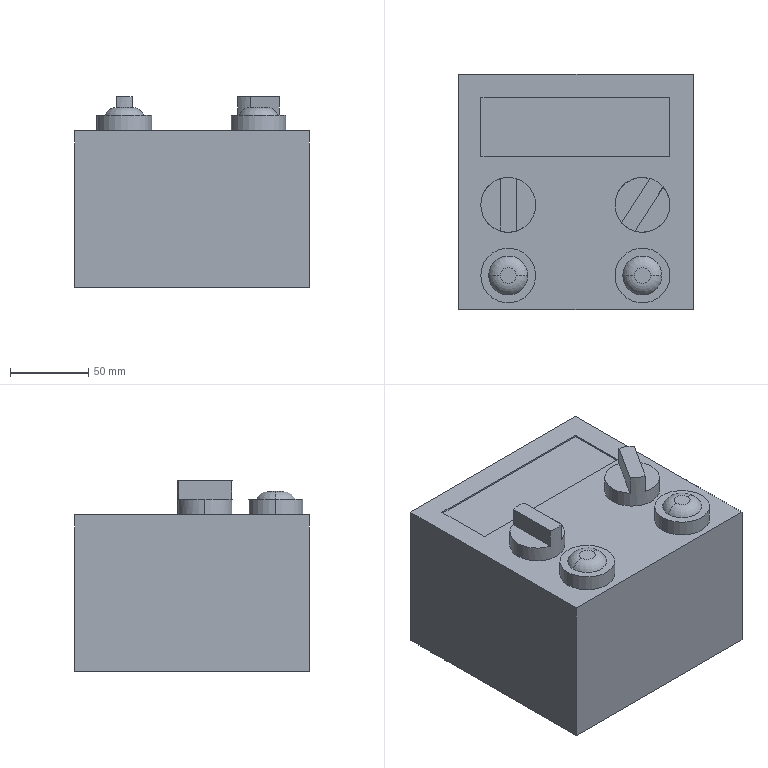Component | SolidWorks | Part2^CentrifugalDehydrator-1 | 1 solid | 44 faces | volume 1195804 mm3 | plane 30 | cylinder 10 | torus 4 | commonest cylinder face diameters 35 x8 20 x2